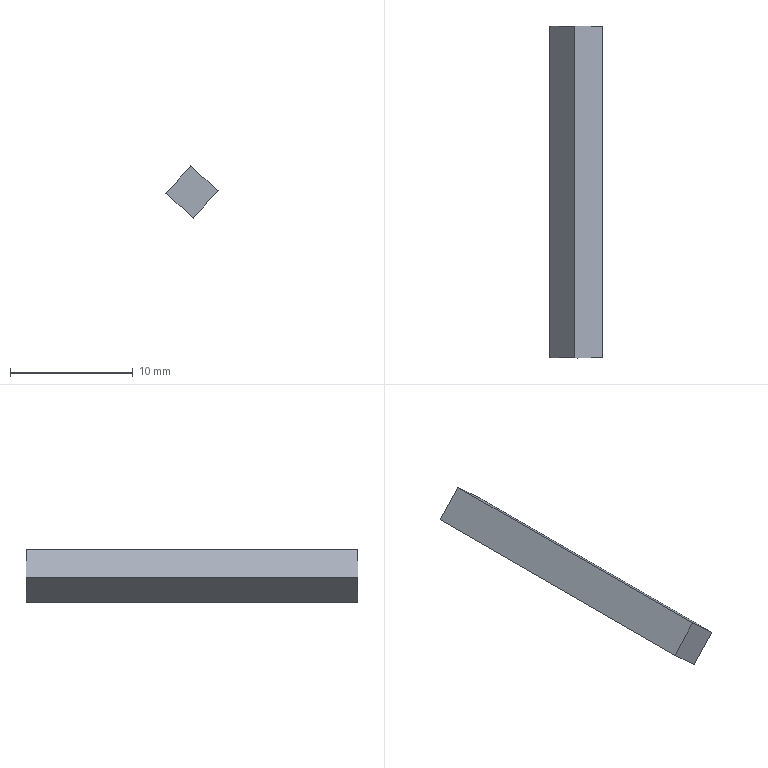Component | SolidWorks | Axe-1 | 1 solid | 6 faces | box 4.24 x 27 x 4.24 mm | volume 243 mm3 | plane 6
STEP:
#1=COLOUR_RGB('',0.7922,0.8196,0.9333);
#2=FILL_AREA_STYLE_COLOUR('',#1);
#3=FILL_AREA_STYLE('',(#2));
#4=SURFACE_STYLE_FILL_AREA(#3);
#5=SURFACE_SIDE_STYLE('',(#4));
#6=SURFACE_STYLE_USAGE(.BOTH.,#5);
#7=PRESENTATION_STYLE_ASSIGNMENT((#6));
#8=CARTESIAN_POINT('',(2.634,2.272,-1.882));
#9=VERTEX_POINT('',#8);
#10=CARTESIAN_POINT('',(2.547,2.272,-1.802));
#11=VERTEX_POINT('',#10);
#12=CARTESIAN_POINT('',(2.547,2.272,-1.802));
#13=DIRECTION('',(-0.7356,0.,0.6774));
#14=VECTOR('',#13,39.37);
#15=LINE('',#12,#14);
#16=EDGE_CURVE('',#9,#11,#15,.T.);
#17=ORIENTED_EDGE('',*,*,#16,.T.);
#18=CARTESIAN_POINT('',(2.547,3.335,-1.802));
#19=VERTEX_POINT('',#18);
#20=CARTESIAN_POINT('',(2.547,3.335,-1.802));
#21=DIRECTION('',(-0.,-1.,-0.));
#22=VECTOR('',#21,39.37);
#23=LINE('',#20,#22);
#24=EDGE_CURVE('',#19,#11,#23,.T.);
#25=ORIENTED_EDGE('',*,*,#24,.F.);
#26=CARTESIAN_POINT('',(2.634,3.335,-1.882));
#27=VERTEX_POINT('',#26);
#28=CARTESIAN_POINT('',(2.547,3.335,-1.802));
#29=DIRECTION('',(-0.7356,0.,0.6774));
#30=VECTOR('',#29,39.37);
#31=LINE('',#28,#30);
#32=EDGE_CURVE('',#27,#19,#31,.T.);
#33=ORIENTED_EDGE('',*,*,#32,.F.);
#34=CARTESIAN_POINT('',(2.634,3.335,-1.882));
#35=DIRECTION('',(-0.,-1.,-0.));
#36=VECTOR('',#35,39.37);
#37=LINE('',#34,#36);
#38=EDGE_CURVE('',#27,#9,#37,.T.);
#39=ORIENTED_EDGE('',*,*,#38,.T.);
#40=EDGE_LOOP('',(#17,#25,#33,#39));
#41=FACE_OUTER_BOUND('',#40,.T.);
#42=CARTESIAN_POINT('',(2.547,3.335,-1.802));
#43=DIRECTION('',(0.6774,-0.,0.7356));
#44=DIRECTION('',(0.7356,-0.,-0.6774));
#45=AXIS2_PLACEMENT_3D('',#42,#43,#44);
#46=PLANE('',#45);
#47=ADVANCED_FACE('',(#41),#46,.F.);
#48=CARTESIAN_POINT('',(2.627,2.272,-1.715));
#49=VERTEX_POINT('',#48);
#50=CARTESIAN_POINT('',(2.627,2.272,-1.715));
#51=DIRECTION('',(0.6774,-0.,0.7356));
#52=VECTOR('',#51,39.37);
#53=LINE('',#50,#52);
#54=EDGE_CURVE('',#11,#49,#53,.T.);
#55=ORIENTED_EDGE('',*,*,#54,.T.);
#56=CARTESIAN_POINT('',(2.627,3.335,-1.715));
#57=VERTEX_POINT('',#56);
#58=CARTESIAN_POINT('',(2.627,3.335,-1.715));
#59=DIRECTION('',(-0.,-1.,-0.));
#60=VECTOR('',#59,39.37);
#61=LINE('',#58,#60);
#62=EDGE_CURVE('',#57,#49,#61,.T.);
#63=ORIENTED_EDGE('',*,*,#62,.F.);
#64=CARTESIAN_POINT('',(2.627,3.335,-1.715));
#65=DIRECTION('',(0.6774,-0.,0.7356));
#66=VECTOR('',#65,39.37);
#67=LINE('',#64,#66);
#68=EDGE_CURVE('',#19,#57,#67,.T.);
#69=ORIENTED_EDGE('',*,*,#68,.F.);
#70=ORIENTED_EDGE('',*,*,#24,.T.);
#71=EDGE_LOOP('',(#55,#63,#69,#70));
#72=FACE_OUTER_BOUND('',#71,.T.);
#73=CARTESIAN_POINT('',(2.627,3.335,-1.715));
#74=DIRECTION('',(0.7356,-0.,-0.6774));
#75=DIRECTION('',(-0.,-1.,-0.));
#76=AXIS2_PLACEMENT_3D('',#73,#74,#75);
#77=PLANE('',#76);
#78=ADVANCED_FACE('',(#72),#77,.F.);
#79=CARTESIAN_POINT('',(2.714,2.272,-1.795));
#80=VERTEX_POINT('',#79);
#81=CARTESIAN_POINT('',(2.627,2.272,-1.715));
#82=DIRECTION('',(0.7356,-0.,-0.6774));
#83=VECTOR('',#82,39.37);
#84=LINE('',#81,#83);
#85=EDGE_CURVE('',#49,#80,#84,.T.);
#86=ORIENTED_EDGE('',*,*,#85,.T.);
#87=CARTESIAN_POINT('',(2.714,3.335,-1.795));
#88=VERTEX_POINT('',#87);
#89=CARTESIAN_POINT('',(2.714,3.335,-1.795));
#90=DIRECTION('',(-0.,-1.,-0.));
#91=VECTOR('',#90,39.37);
#92=LINE('',#89,#91);
#93=EDGE_CURVE('',#88,#80,#92,.T.);
#94=ORIENTED_EDGE('',*,*,#93,.F.);
#95=CARTESIAN_POINT('',(2.627,3.335,-1.715));
#96=DIRECTION('',(0.7356,-0.,-0.6774));
#97=VECTOR('',#96,39.37);
#98=LINE('',#95,#97);
#99=EDGE_CURVE('',#57,#88,#98,.T.);
#100=ORIENTED_EDGE('',*,*,#99,.F.);
#101=ORIENTED_EDGE('',*,*,#62,.T.);
#102=EDGE_LOOP('',(#86,#94,#100,#101));
#103=FACE_OUTER_BOUND('',#102,.T.);
#104=CARTESIAN_POINT('',(2.627,3.335,-1.715));
#105=DIRECTION('',(-0.6774,0.,-0.7356));
#106=DIRECTION('',(-0.7356,0.,0.6774));
#107=AXIS2_PLACEMENT_3D('',#104,#105,#106);
#108=PLANE('',#107);
#109=ADVANCED_FACE('',(#103),#108,.F.);
#110=CARTESIAN_POINT('',(2.714,2.272,-1.795));
#111=DIRECTION('',(-0.6774,0.,-0.7356));
#112=VECTOR('',#111,39.37);
#113=LINE('',#110,#112);
#114=EDGE_CURVE('',#80,#9,#113,.T.);
#115=ORIENTED_EDGE('',*,*,#114,.T.);
#116=ORIENTED_EDGE('',*,*,#38,.F.);
#117=CARTESIAN_POINT('',(2.714,3.335,-1.795));
#118=DIRECTION('',(-0.6774,0.,-0.7356));
#119=VECTOR('',#118,39.37);
#120=LINE('',#117,#119);
#121=EDGE_CURVE('',#88,#27,#120,.T.);
#122=ORIENTED_EDGE('',*,*,#121,.F.);
#123=ORIENTED_EDGE('',*,*,#93,.T.);
#124=EDGE_LOOP('',(#115,#116,#122,#123));
#125=FACE_OUTER_BOUND('',#124,.T.);
#126=CARTESIAN_POINT('',(2.714,3.335,-1.795));
#127=DIRECTION('',(-0.7356,0.,0.6774));
#128=DIRECTION('',(0.,1.,0.));
#129=AXIS2_PLACEMENT_3D('',#126,#127,#128);
#130=PLANE('',#129);
#131=ADVANCED_FACE('',(#125),#130,.F.);
#132=ORIENTED_EDGE('',*,*,#32,.T.);
#133=ORIENTED_EDGE('',*,*,#68,.T.);
#134=ORIENTED_EDGE('',*,*,#99,.T.);
#135=ORIENTED_EDGE('',*,*,#121,.T.);
#136=EDGE_LOOP('',(#132,#133,#134,#135));
#137=FACE_OUTER_BOUND('',#136,.T.);
#138=CARTESIAN_POINT('',(2.63,3.335,-1.799));
#139=DIRECTION('',(0.,1.,0.));
#140=DIRECTION('',(-0.6774,0.,-0.7356));
#141=AXIS2_PLACEMENT_3D('',#138,#139,#140);
#142=PLANE('',#141);
#143=ADVANCED_FACE('',(#137),#142,.T.);
#144=ORIENTED_EDGE('',*,*,#16,.F.);
#145=ORIENTED_EDGE('',*,*,#114,.F.);
#146=ORIENTED_EDGE('',*,*,#85,.F.);
#147=ORIENTED_EDGE('',*,*,#54,.F.);
#148=EDGE_LOOP('',(#144,#145,#146,#147));
#149=FACE_OUTER_BOUND('',#148,.T.);
#150=CARTESIAN_POINT('',(2.63,2.272,-1.799));
#151=DIRECTION('',(0.,1.,0.));
#152=DIRECTION('',(-0.6774,0.,-0.7356));
#153=AXIS2_PLACEMENT_3D('',#150,#151,#152);
#154=PLANE('',#153);
#155=ADVANCED_FACE('',(#149),#154,.F.);
#156=CLOSED_SHELL('',(#47,#78,#109,#131,#143,#155));
#157=MANIFOLD_SOLID_BREP('',#156);
#158=STYLED_ITEM('',(#7),#157);
#159=(LENGTH_UNIT()NAMED_UNIT(*)SI_UNIT($,.METRE.));
#160=LENGTH_MEASURE_WITH_UNIT(LENGTH_MEASURE(0.0254),#159);
#161=DIMENSIONAL_EXPONENTS(1.,0.,0.,0.,0.,0.,0.);
#162=(CONVERSION_BASED_UNIT('',#160)LENGTH_UNIT()NAMED_UNIT(#161));
#163=UNCERTAINTY_MEASURE_WITH_UNIT(LENGTH_MEASURE(0.00001),#162,'','');
#164=(NAMED_UNIT(*)PLANE_ANGLE_UNIT()SI_UNIT($,.RADIAN.));
#165=(NAMED_UNIT(*)SI_UNIT($,.STERADIAN.)SOLID_ANGLE_UNIT());
#166=(GEOMETRIC_REPRESENTATION_CONTEXT(3)GLOBAL_UNCERTAINTY_ASSIGNED_CONTEXT((#163))GLOBAL_UNIT_ASSIGNED_CONTEXT((#162,#164,#165))REPRESENTATION_CONTEXT('',''));
#167=MECHANICAL_DESIGN_GEOMETRIC_PRESENTATION_REPRESENTATION('',(#158),#166);
#168=PRESENTATION_LAYER_ASSIGNMENT('','',(#158));
#169=CARTESIAN_POINT('',(0.,0.,0.));
#170=DIRECTION('',(0.,0.,1.));
#171=DIRECTION('',(1.,0.,0.));
#172=AXIS2_PLACEMENT_3D('',#169,#170,#171);
#173=(LENGTH_UNIT()NAMED_UNIT(*)SI_UNIT($,.METRE.));
#174=LENGTH_MEASURE_WITH_UNIT(LENGTH_MEASURE(0.0254),#173);
#175=DIMENSIONAL_EXPONENTS(1.,0.,0.,0.,0.,0.,0.);
#176=(CONVERSION_BASED_UNIT('',#174)LENGTH_UNIT()NAMED_UNIT(#175));
#177=UNCERTAINTY_MEASURE_WITH_UNIT(LENGTH_MEASURE(0.00001),#176,'','');
#178=(NAMED_UNIT(*)PLANE_ANGLE_UNIT()SI_UNIT($,.RADIAN.));
#179=(NAMED_UNIT(*)SI_UNIT($,.STERADIAN.)SOLID_ANGLE_UNIT());
#180=(GEOMETRIC_REPRESENTATION_CONTEXT(3)GLOBAL_UNCERTAINTY_ASSIGNED_CONTEXT((#177))GLOBAL_UNIT_ASSIGNED_CONTEXT((#176,#178,#179))REPRESENTATION_CONTEXT('',''));
#181=ADVANCED_BREP_SHAPE_REPRESENTATION('',(#157,#172),#180);